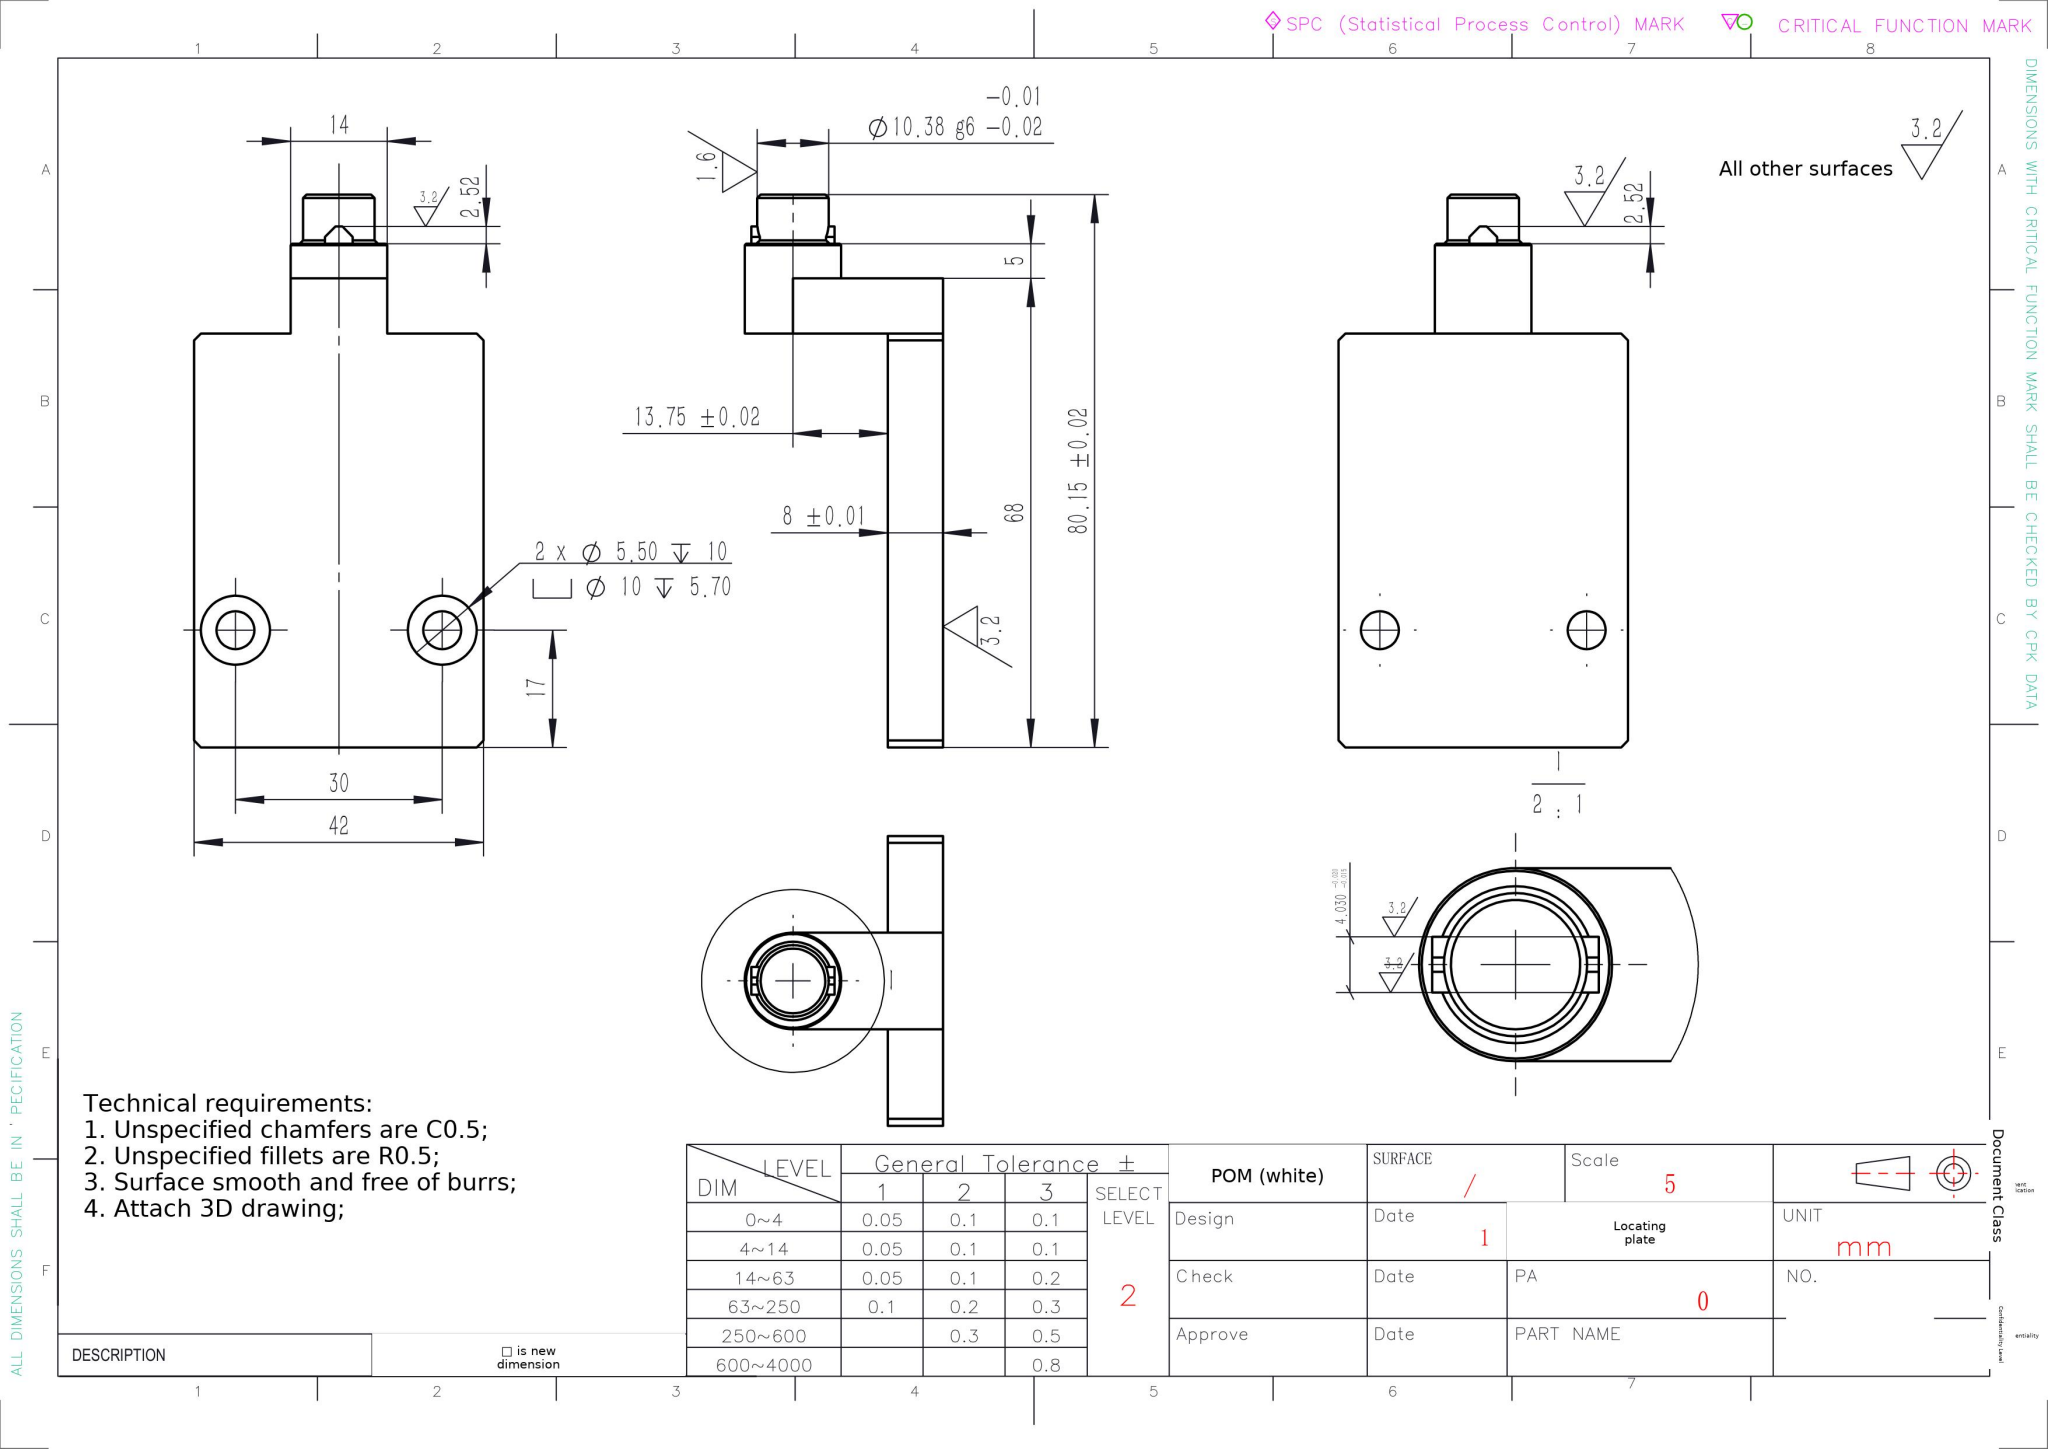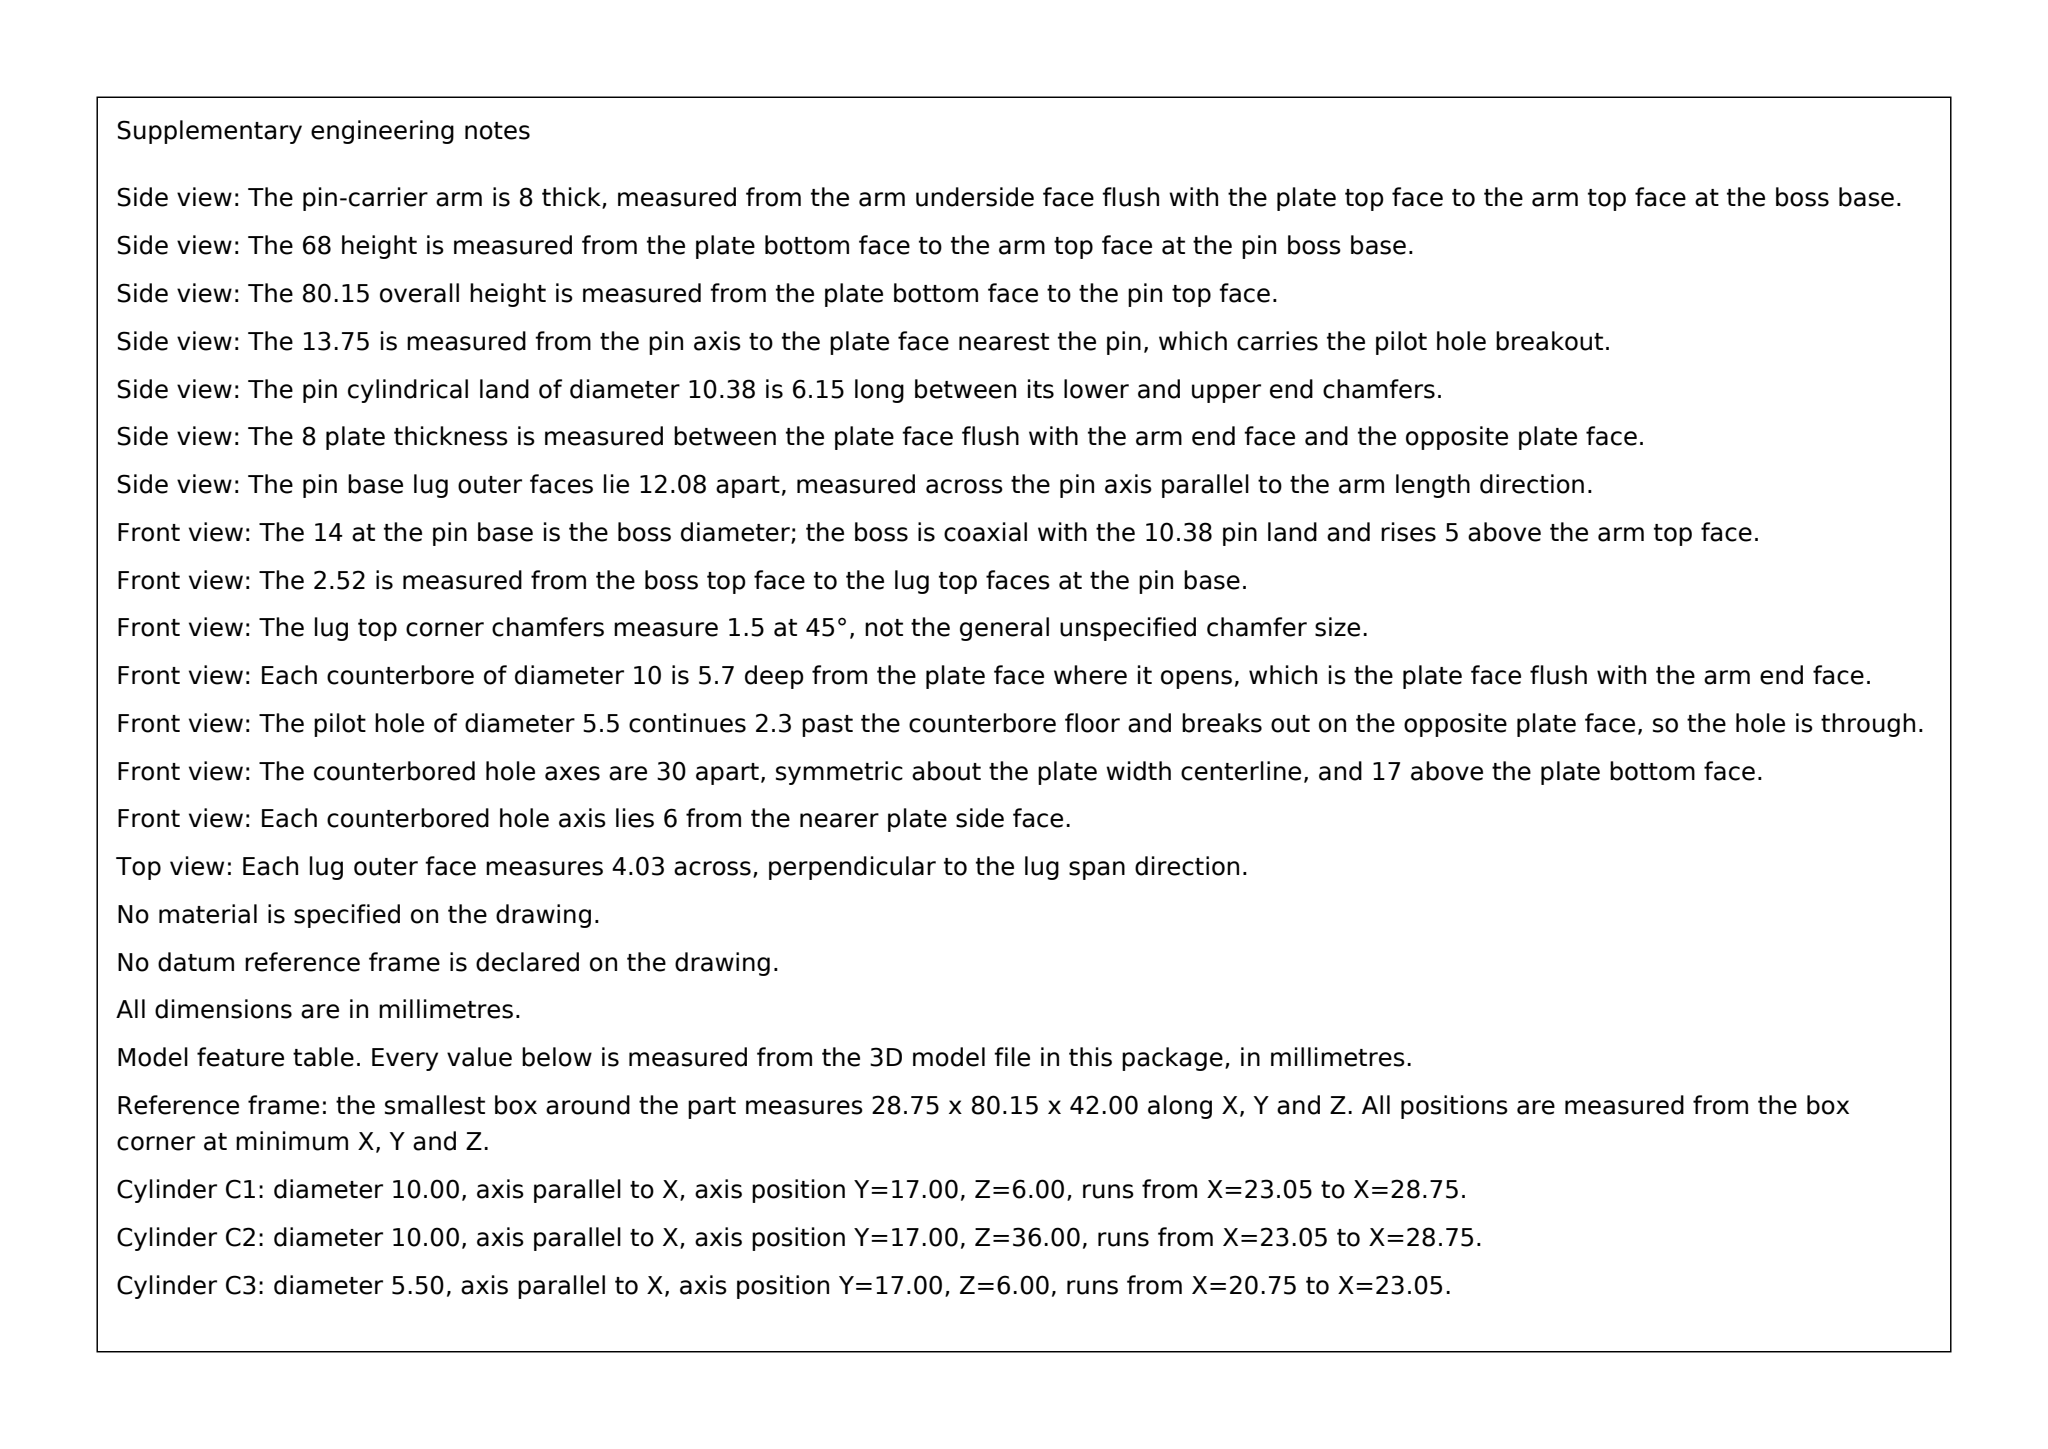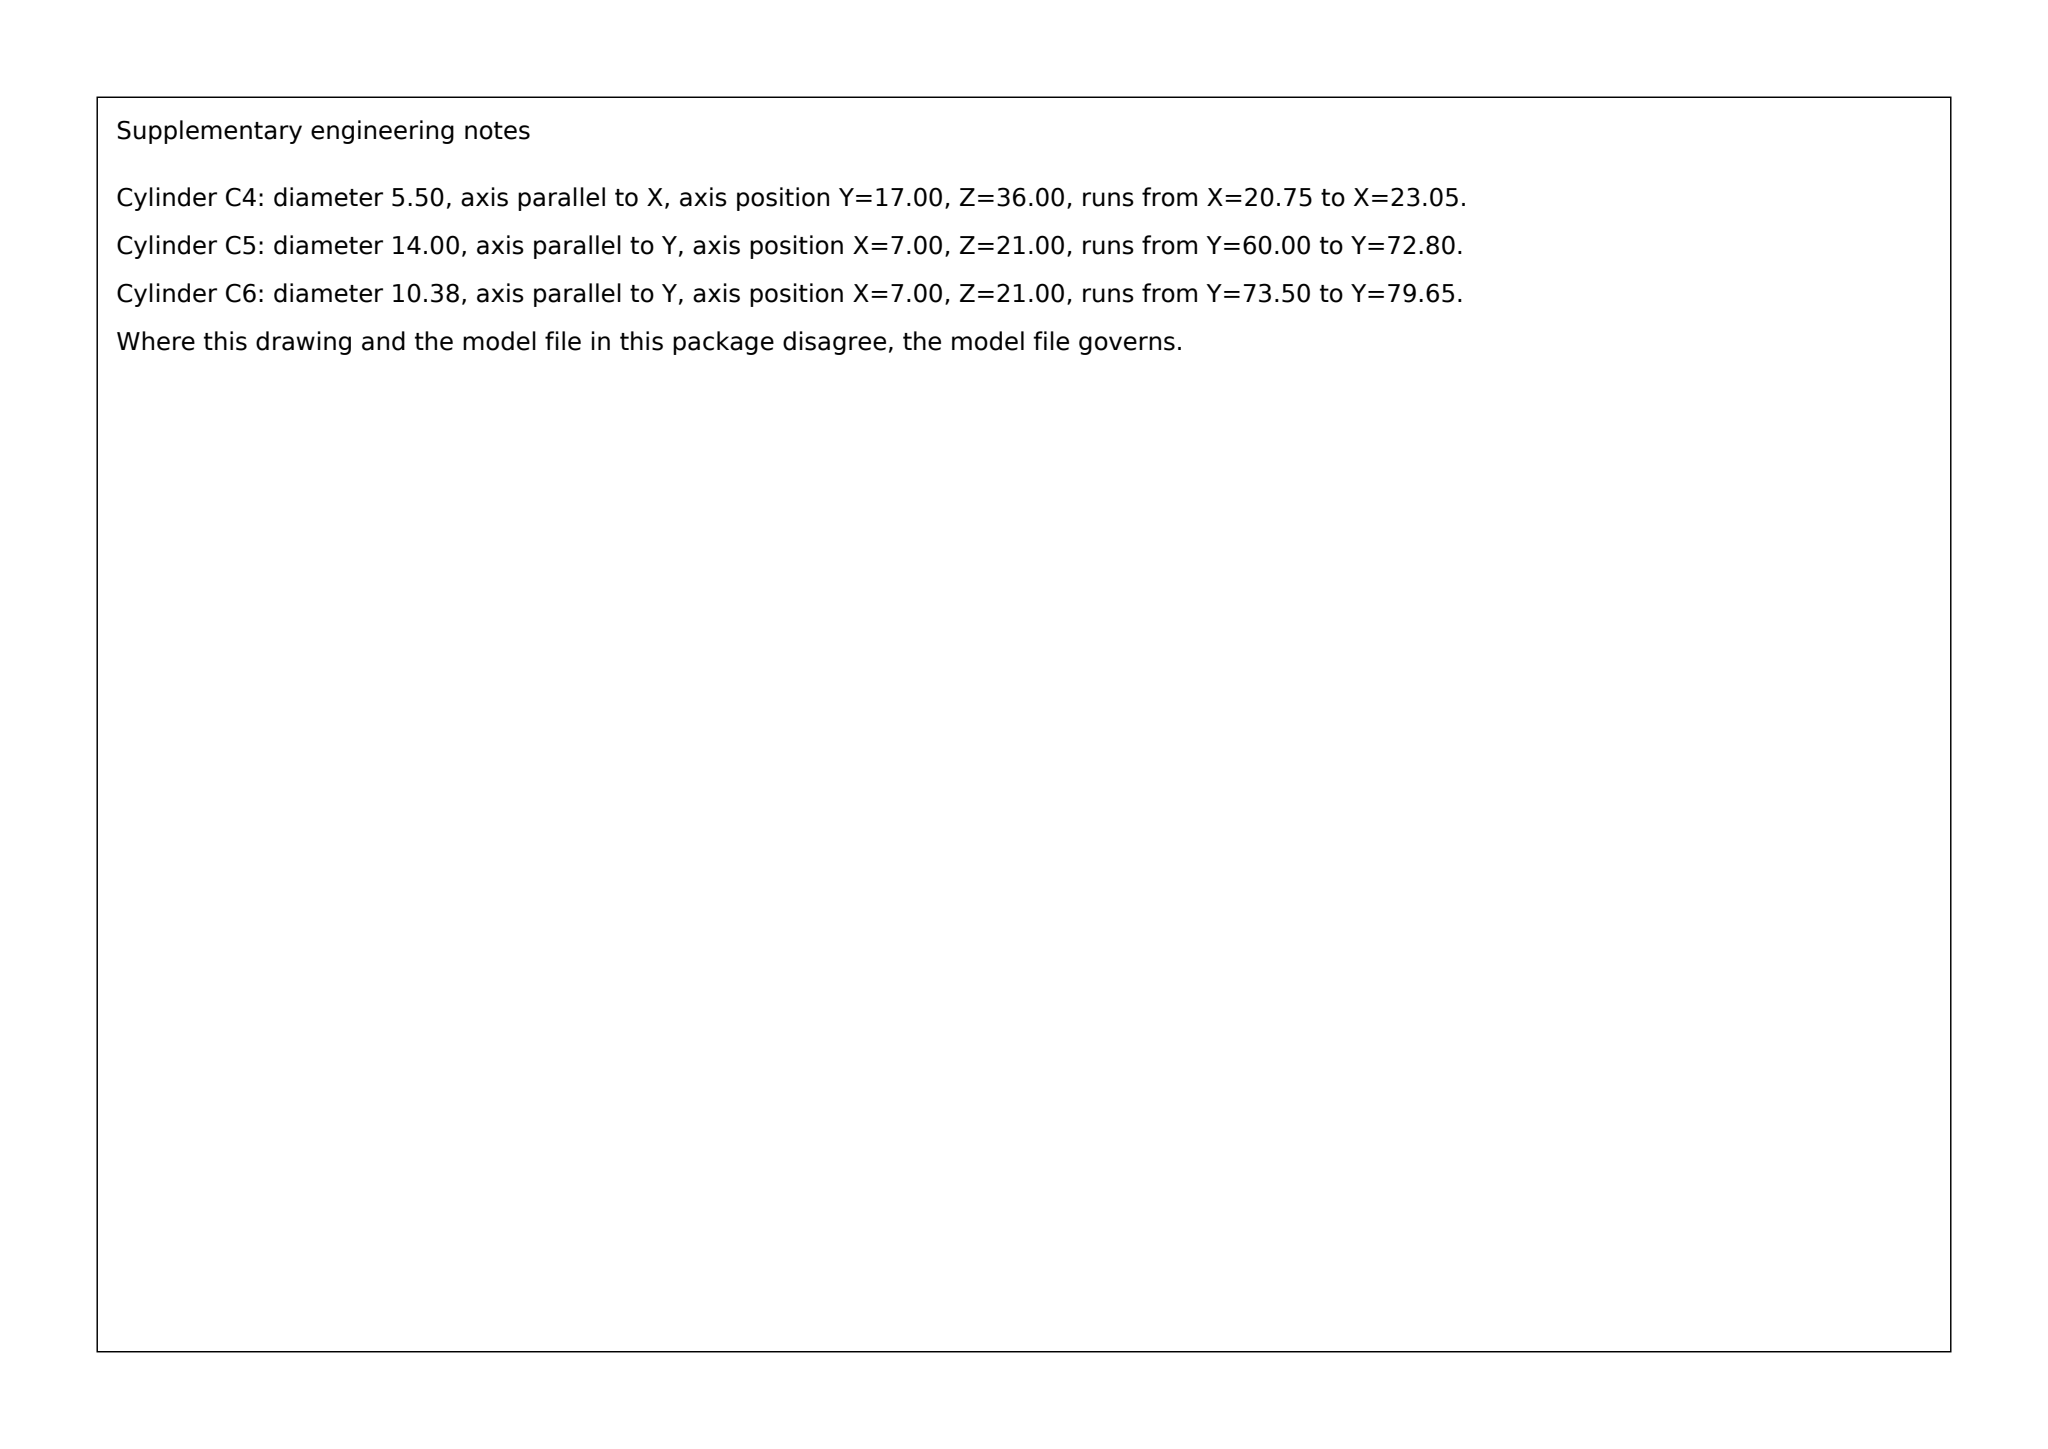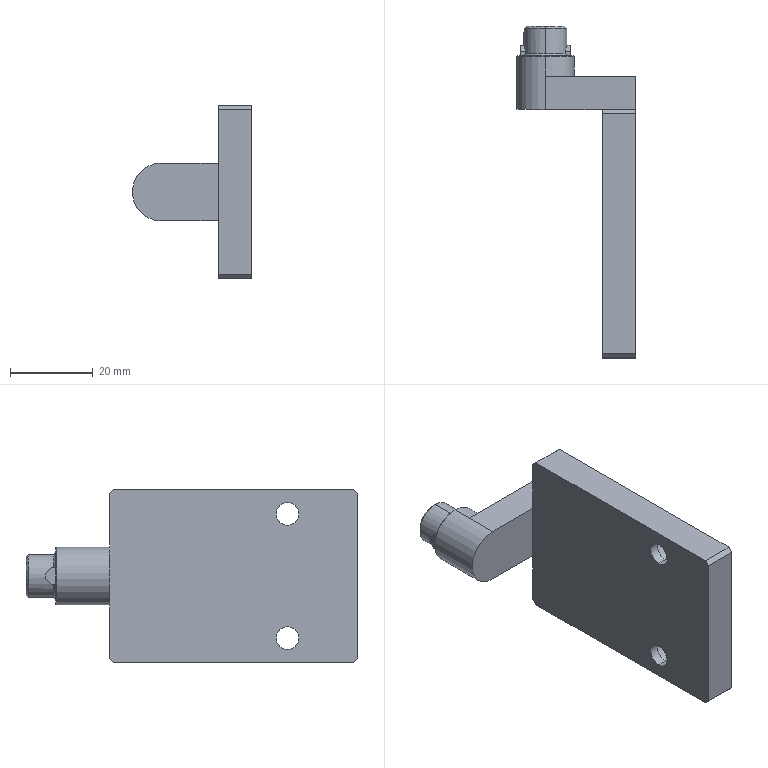Part | SolidWorks | mm | material pom | 1 solid | 50 faces | box 28.75 x 80.15 x 42 mm | volume 23579 mm3 | plane 31 | cylinder 12 | cone 7 | commonest cylinder face diameters 10 x4 5.5 x4 10.38 x2 14 x2
Drawing notes:
SLOT IN Ø14 BOSS: 4.03 WIDE x 12.08 LG, CTRD ON PIN AXIS | from the solid: x-planes 0.96 & 13.04 (12.08 apart, sym about boss axis x=7); slot width 4.030
42 WIDE BODY: 60 FROM BOTTOM TO 14 WIDE NECK STEP (NECK 8 LG) | from the solid: y-planes 0, 60 (step face), 68 (neck top); 68-60=8
Ø14 BOSS END: C0.2 x 45° TO Ø13.6 | from the solid: cone 90° incl, ref dia 13.60 on Ø14 boss end